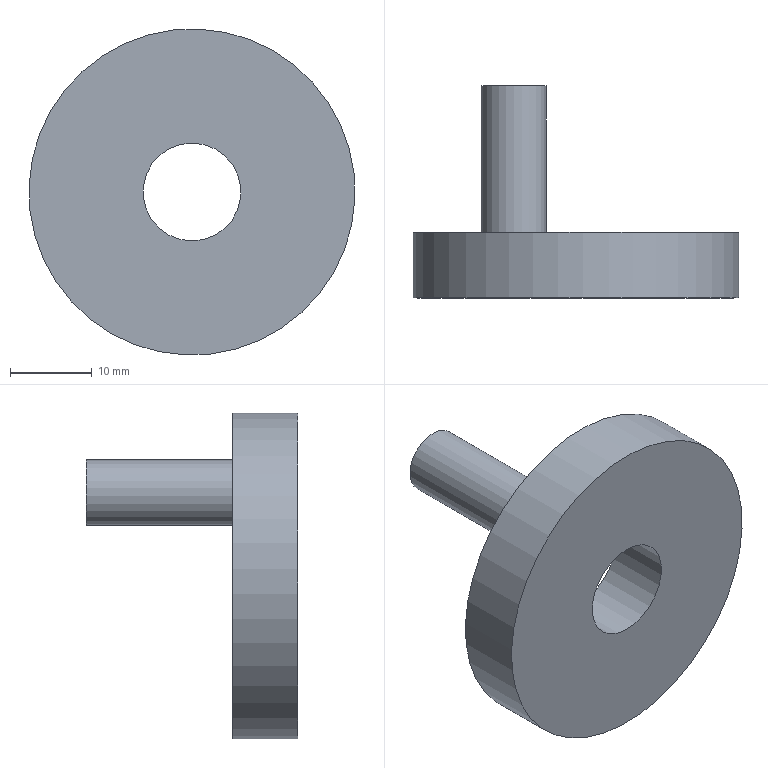Component | NX | CRANK | 1 solid | 6 faces | box 40 x 26 x 40 mm | volume 10053 mm3 | cylinder 3 | plane 3 | commonest cylinder face diameters 40 x1 12 x1 8 x1
STEP:
#1=CARTESIAN_POINT('',(0.,0.,0.));
#2=DIRECTION('',(0.,0.,1.));
#3=DIRECTION('',(1.,0.,0.));
#4=AXIS2_PLACEMENT_3D('',#1,#2,#3);
#5=CARTESIAN_POINT('',(-19.874,30.,-2.24));
#6=VERTEX_POINT('',#5);
#7=CARTESIAN_POINT('',(-0.,30.,0.));
#8=DIRECTION('',(0.,1.,0.));
#9=DIRECTION('',(-0.9937,0.,-0.112));
#10=AXIS2_PLACEMENT_3D('',#7,#8,#9);
#11=CIRCLE('',#10,20.);
#12=CARTESIAN_POINT('',(-0.,30.,0.));
#13=DIRECTION('',(0.,-1.,0.));
#14=DIRECTION('',(0.9937,0.,0.112));
#15=AXIS2_PLACEMENT_3D('',#12,#13,#14);
#16=CYLINDRICAL_SURFACE('',#15,20.);
#17=CARTESIAN_POINT('',(9.425,0.));
#18=DIRECTION('',(-1.,0.));
#19=VECTOR('',#18,1.);
#20=LINE('',#17,#19);
#21=(GEOMETRIC_REPRESENTATION_CONTEXT(2)PARAMETRIC_REPRESENTATION_CONTEXT()REPRESENTATION_CONTEXT('',''));
#22=DEFINITIONAL_REPRESENTATION('',(#20),#21);
#23=PCURVE('',#16,#22);
#24=CARTESIAN_POINT('',(-0.,30.,0.));
#25=DIRECTION('',(0.,1.,0.));
#26=DIRECTION('',(-0.9937,0.,-0.112));
#27=AXIS2_PLACEMENT_3D('',#24,#25,#26);
#28=PLANE('',#27);
#29=CARTESIAN_POINT('',(0.,0.));
#30=DIRECTION('',(1.,0.));
#31=AXIS2_PLACEMENT_2D('',#29,#30);
#32=CIRCLE('',#31,20.);
#33=(GEOMETRIC_REPRESENTATION_CONTEXT(2)PARAMETRIC_REPRESENTATION_CONTEXT()REPRESENTATION_CONTEXT('',''));
#34=DEFINITIONAL_REPRESENTATION('',(#32),#33);
#35=PCURVE('',#28,#34);
#36=SURFACE_CURVE('',#11,(#23,#35),.PCURVE_S1.);
#37=EDGE_CURVE('',#6,#6,#36,.T.);
#38=ORIENTED_EDGE('',*,*,#37,.F.);
#39=CARTESIAN_POINT('',(-19.874,22.,-2.24));
#40=VERTEX_POINT('',#39);
#41=CARTESIAN_POINT('',(-19.874,30.,-2.24));
#42=CARTESIAN_POINT('',(-19.874,22.,-2.24));
#43=B_SPLINE_CURVE_WITH_KNOTS('',1,(#41,#42),.UNSPECIFIED.,.F.,.F.,(2,2),(0.,8.),.PIECEWISE_BEZIER_KNOTS.);
#44=CARTESIAN_POINT('',(9.425,0.));
#45=DIRECTION('',(0.,1.));
#46=VECTOR('',#45,1.);
#47=LINE('',#44,#46);
#48=(GEOMETRIC_REPRESENTATION_CONTEXT(2)PARAMETRIC_REPRESENTATION_CONTEXT()REPRESENTATION_CONTEXT('',''));
#49=DEFINITIONAL_REPRESENTATION('',(#47),#48);
#50=PCURVE('',#16,#49);
#51=CARTESIAN_POINT('',(3.142,0.));
#52=DIRECTION('',(0.,1.));
#53=VECTOR('',#52,1.);
#54=LINE('',#51,#53);
#55=(GEOMETRIC_REPRESENTATION_CONTEXT(2)PARAMETRIC_REPRESENTATION_CONTEXT()REPRESENTATION_CONTEXT('',''));
#56=DEFINITIONAL_REPRESENTATION('',(#54),#55);
#57=PCURVE('',#16,#56);
#58=SEAM_CURVE('',#43,(#50,#57),.PCURVE_S1.);
#59=EDGE_CURVE('',#6,#40,#58,.T.);
#60=ORIENTED_EDGE('',*,*,#59,.T.);
#61=CARTESIAN_POINT('',(-0.,22.,0.));
#62=DIRECTION('',(0.,1.,0.));
#63=DIRECTION('',(-0.9937,0.,-0.112));
#64=AXIS2_PLACEMENT_3D('',#61,#62,#63);
#65=CIRCLE('',#64,20.);
#66=CARTESIAN_POINT('',(9.425,8.));
#67=DIRECTION('',(-1.,0.));
#68=VECTOR('',#67,1.);
#69=LINE('',#66,#68);
#70=(GEOMETRIC_REPRESENTATION_CONTEXT(2)PARAMETRIC_REPRESENTATION_CONTEXT()REPRESENTATION_CONTEXT('',''));
#71=DEFINITIONAL_REPRESENTATION('',(#69),#70);
#72=PCURVE('',#16,#71);
#73=CARTESIAN_POINT('',(-0.,22.,0.));
#74=DIRECTION('',(0.,1.,0.));
#75=DIRECTION('',(-0.9937,0.,-0.112));
#76=AXIS2_PLACEMENT_3D('',#73,#74,#75);
#77=PLANE('',#76);
#78=CARTESIAN_POINT('',(0.,0.));
#79=DIRECTION('',(1.,0.));
#80=AXIS2_PLACEMENT_2D('',#78,#79);
#81=CIRCLE('',#80,20.);
#82=(GEOMETRIC_REPRESENTATION_CONTEXT(2)PARAMETRIC_REPRESENTATION_CONTEXT()REPRESENTATION_CONTEXT('',''));
#83=DEFINITIONAL_REPRESENTATION('',(#81),#82);
#84=PCURVE('',#77,#83);
#85=SURFACE_CURVE('',#65,(#72,#84),.PCURVE_S1.);
#86=EDGE_CURVE('',#40,#40,#85,.T.);
#87=ORIENTED_EDGE('',*,*,#86,.T.);
#88=ORIENTED_EDGE('',*,*,#59,.F.);
#89=EDGE_LOOP('',(#38,#60,#87,#88));
#90=FACE_BOUND('',#89,.T.);
#91=ADVANCED_FACE('',(#90),#16,.T.);
#92=CARTESIAN_POINT('',(-5.962,30.,-0.672));
#93=VERTEX_POINT('',#92);
#94=CARTESIAN_POINT('',(-0.,30.,0.));
#95=DIRECTION('',(0.,1.,0.));
#96=DIRECTION('',(-0.9937,0.,-0.112));
#97=AXIS2_PLACEMENT_3D('',#94,#95,#96);
#98=CIRCLE('',#97,6.);
#99=CARTESIAN_POINT('',(-0.,30.,0.));
#100=DIRECTION('',(0.,-1.,0.));
#101=DIRECTION('',(0.9937,0.,0.112));
#102=AXIS2_PLACEMENT_3D('',#99,#100,#101);
#103=CYLINDRICAL_SURFACE('',#102,6.);
#104=CARTESIAN_POINT('',(9.425,0.));
#105=DIRECTION('',(-1.,0.));
#106=VECTOR('',#105,1.);
#107=LINE('',#104,#106);
#108=(GEOMETRIC_REPRESENTATION_CONTEXT(2)PARAMETRIC_REPRESENTATION_CONTEXT()REPRESENTATION_CONTEXT('',''));
#109=DEFINITIONAL_REPRESENTATION('',(#107),#108);
#110=PCURVE('',#103,#109);
#111=CARTESIAN_POINT('',(0.,0.));
#112=DIRECTION('',(1.,0.));
#113=AXIS2_PLACEMENT_2D('',#111,#112);
#114=CIRCLE('',#113,6.);
#115=(GEOMETRIC_REPRESENTATION_CONTEXT(2)PARAMETRIC_REPRESENTATION_CONTEXT()REPRESENTATION_CONTEXT('',''));
#116=DEFINITIONAL_REPRESENTATION('',(#114),#115);
#117=PCURVE('',#28,#116);
#118=SURFACE_CURVE('',#98,(#110,#117),.PCURVE_S1.);
#119=EDGE_CURVE('',#93,#93,#118,.T.);
#120=ORIENTED_EDGE('',*,*,#119,.F.);
#121=CARTESIAN_POINT('',(-5.962,22.,-0.672));
#122=VERTEX_POINT('',#121);
#123=CARTESIAN_POINT('',(-5.962,30.,-0.672));
#124=CARTESIAN_POINT('',(-5.962,22.,-0.672));
#125=B_SPLINE_CURVE_WITH_KNOTS('',1,(#123,#124),.UNSPECIFIED.,.F.,.F.,(2,2),(0.,8.),.PIECEWISE_BEZIER_KNOTS.);
#126=CARTESIAN_POINT('',(9.425,0.));
#127=DIRECTION('',(0.,1.));
#128=VECTOR('',#127,1.);
#129=LINE('',#126,#128);
#130=(GEOMETRIC_REPRESENTATION_CONTEXT(2)PARAMETRIC_REPRESENTATION_CONTEXT()REPRESENTATION_CONTEXT('',''));
#131=DEFINITIONAL_REPRESENTATION('',(#129),#130);
#132=PCURVE('',#103,#131);
#133=CARTESIAN_POINT('',(3.142,0.));
#134=DIRECTION('',(0.,1.));
#135=VECTOR('',#134,1.);
#136=LINE('',#133,#135);
#137=(GEOMETRIC_REPRESENTATION_CONTEXT(2)PARAMETRIC_REPRESENTATION_CONTEXT()REPRESENTATION_CONTEXT('',''));
#138=DEFINITIONAL_REPRESENTATION('',(#136),#137);
#139=PCURVE('',#103,#138);
#140=SEAM_CURVE('',#125,(#132,#139),.PCURVE_S1.);
#141=EDGE_CURVE('',#93,#122,#140,.T.);
#142=ORIENTED_EDGE('',*,*,#141,.T.);
#143=CARTESIAN_POINT('',(-0.,22.,0.));
#144=DIRECTION('',(0.,1.,0.));
#145=DIRECTION('',(-0.9937,0.,-0.112));
#146=AXIS2_PLACEMENT_3D('',#143,#144,#145);
#147=CIRCLE('',#146,6.);
#148=CARTESIAN_POINT('',(9.425,8.));
#149=DIRECTION('',(-1.,0.));
#150=VECTOR('',#149,1.);
#151=LINE('',#148,#150);
#152=(GEOMETRIC_REPRESENTATION_CONTEXT(2)PARAMETRIC_REPRESENTATION_CONTEXT()REPRESENTATION_CONTEXT('',''));
#153=DEFINITIONAL_REPRESENTATION('',(#151),#152);
#154=PCURVE('',#103,#153);
#155=CARTESIAN_POINT('',(0.,0.));
#156=DIRECTION('',(1.,0.));
#157=AXIS2_PLACEMENT_2D('',#155,#156);
#158=CIRCLE('',#157,6.);
#159=(GEOMETRIC_REPRESENTATION_CONTEXT(2)PARAMETRIC_REPRESENTATION_CONTEXT()REPRESENTATION_CONTEXT('',''));
#160=DEFINITIONAL_REPRESENTATION('',(#158),#159);
#161=PCURVE('',#77,#160);
#162=SURFACE_CURVE('',#147,(#154,#161),.PCURVE_S1.);
#163=EDGE_CURVE('',#122,#122,#162,.T.);
#164=ORIENTED_EDGE('',*,*,#163,.T.);
#165=ORIENTED_EDGE('',*,*,#141,.F.);
#166=EDGE_LOOP('',(#120,#142,#164,#165));
#167=FACE_BOUND('',#166,.F.);
#168=ADVANCED_FACE('',(#167),#103,.F.);
#169=CARTESIAN_POINT('',(-11.615,30.,9.787));
#170=VERTEX_POINT('',#169);
#171=CARTESIAN_POINT('',(-7.64,30.,10.235));
#172=DIRECTION('',(0.,1.,0.));
#173=DIRECTION('',(-0.9937,0.,-0.112));
#174=AXIS2_PLACEMENT_3D('',#171,#172,#173);
#175=CIRCLE('',#174,4.);
#176=CARTESIAN_POINT('',(6.446,11.027));
#177=DIRECTION('',(1.,0.));
#178=AXIS2_PLACEMENT_2D('',#176,#177);
#179=CIRCLE('',#178,4.);
#180=(GEOMETRIC_REPRESENTATION_CONTEXT(2)PARAMETRIC_REPRESENTATION_CONTEXT()REPRESENTATION_CONTEXT('',''));
#181=DEFINITIONAL_REPRESENTATION('',(#179),#180);
#182=PCURVE('',#28,#181);
#183=CARTESIAN_POINT('',(-7.64,48.,10.235));
#184=DIRECTION('',(0.,-1.,0.));
#185=DIRECTION('',(0.9937,0.,0.112));
#186=AXIS2_PLACEMENT_3D('',#183,#184,#185);
#187=CYLINDRICAL_SURFACE('',#186,4.);
#188=CARTESIAN_POINT('',(9.425,18.));
#189=DIRECTION('',(-1.,0.));
#190=VECTOR('',#189,1.);
#191=LINE('',#188,#190);
#192=(GEOMETRIC_REPRESENTATION_CONTEXT(2)PARAMETRIC_REPRESENTATION_CONTEXT()REPRESENTATION_CONTEXT('',''));
#193=DEFINITIONAL_REPRESENTATION('',(#191),#192);
#194=PCURVE('',#187,#193);
#195=SURFACE_CURVE('',#175,(#182,#194),.PCURVE_S1.);
#196=EDGE_CURVE('',#170,#170,#195,.T.);
#197=ORIENTED_EDGE('',*,*,#196,.F.);
#198=EDGE_LOOP('',(#197));
#199=FACE_BOUND('',#198,.T.);
#200=ORIENTED_EDGE('',*,*,#37,.T.);
#201=EDGE_LOOP('',(#200));
#202=FACE_BOUND('',#201,.T.);
#203=ORIENTED_EDGE('',*,*,#119,.F.);
#204=EDGE_LOOP('',(#203));
#205=FACE_BOUND('',#204,.T.);
#206=ADVANCED_FACE('',(#199,#202,#205),#28,.T.);
#207=ORIENTED_EDGE('',*,*,#86,.F.);
#208=EDGE_LOOP('',(#207));
#209=FACE_BOUND('',#208,.T.);
#210=ORIENTED_EDGE('',*,*,#163,.T.);
#211=EDGE_LOOP('',(#210));
#212=FACE_BOUND('',#211,.T.);
#213=ADVANCED_FACE('',(#209,#212),#77,.F.);
#214=CARTESIAN_POINT('',(-11.615,48.,9.787));
#215=VERTEX_POINT('',#214);
#216=CARTESIAN_POINT('',(-7.64,48.,10.235));
#217=DIRECTION('',(0.,1.,0.));
#218=DIRECTION('',(-0.9937,0.,-0.112));
#219=AXIS2_PLACEMENT_3D('',#216,#217,#218);
#220=CIRCLE('',#219,4.);
#221=CARTESIAN_POINT('',(9.425,0.));
#222=DIRECTION('',(-1.,0.));
#223=VECTOR('',#222,1.);
#224=LINE('',#221,#223);
#225=(GEOMETRIC_REPRESENTATION_CONTEXT(2)PARAMETRIC_REPRESENTATION_CONTEXT()REPRESENTATION_CONTEXT('',''));
#226=DEFINITIONAL_REPRESENTATION('',(#224),#225);
#227=PCURVE('',#187,#226);
#228=CARTESIAN_POINT('',(-7.64,48.,10.235));
#229=DIRECTION('',(0.,1.,0.));
#230=DIRECTION('',(-0.9937,0.,-0.112));
#231=AXIS2_PLACEMENT_3D('',#228,#229,#230);
#232=PLANE('',#231);
#233=CARTESIAN_POINT('',(0.,0.));
#234=DIRECTION('',(1.,0.));
#235=AXIS2_PLACEMENT_2D('',#233,#234);
#236=CIRCLE('',#235,4.);
#237=(GEOMETRIC_REPRESENTATION_CONTEXT(2)PARAMETRIC_REPRESENTATION_CONTEXT()REPRESENTATION_CONTEXT('',''));
#238=DEFINITIONAL_REPRESENTATION('',(#236),#237);
#239=PCURVE('',#232,#238);
#240=SURFACE_CURVE('',#220,(#227,#239),.PCURVE_S1.);
#241=EDGE_CURVE('',#215,#215,#240,.T.);
#242=ORIENTED_EDGE('',*,*,#241,.F.);
#243=CARTESIAN_POINT('',(-11.615,48.,9.787));
#244=CARTESIAN_POINT('',(-11.615,30.,9.787));
#245=B_SPLINE_CURVE_WITH_KNOTS('',1,(#243,#244),.UNSPECIFIED.,.F.,.F.,(2,2),(0.,18.),.PIECEWISE_BEZIER_KNOTS.);
#246=CARTESIAN_POINT('',(9.425,0.));
#247=DIRECTION('',(0.,1.));
#248=VECTOR('',#247,1.);
#249=LINE('',#246,#248);
#250=(GEOMETRIC_REPRESENTATION_CONTEXT(2)PARAMETRIC_REPRESENTATION_CONTEXT()REPRESENTATION_CONTEXT('',''));
#251=DEFINITIONAL_REPRESENTATION('',(#249),#250);
#252=PCURVE('',#187,#251);
#253=CARTESIAN_POINT('',(3.142,0.));
#254=DIRECTION('',(0.,1.));
#255=VECTOR('',#254,1.);
#256=LINE('',#253,#255);
#257=(GEOMETRIC_REPRESENTATION_CONTEXT(2)PARAMETRIC_REPRESENTATION_CONTEXT()REPRESENTATION_CONTEXT('',''));
#258=DEFINITIONAL_REPRESENTATION('',(#256),#257);
#259=PCURVE('',#187,#258);
#260=SEAM_CURVE('',#245,(#252,#259),.PCURVE_S1.);
#261=EDGE_CURVE('',#215,#170,#260,.T.);
#262=ORIENTED_EDGE('',*,*,#261,.T.);
#263=ORIENTED_EDGE('',*,*,#196,.T.);
#264=ORIENTED_EDGE('',*,*,#261,.F.);
#265=EDGE_LOOP('',(#242,#262,#263,#264));
#266=FACE_BOUND('',#265,.T.);
#267=ADVANCED_FACE('',(#266),#187,.T.);
#268=ORIENTED_EDGE('',*,*,#241,.T.);
#269=EDGE_LOOP('',(#268));
#270=FACE_BOUND('',#269,.T.);
#271=ADVANCED_FACE('',(#270),#232,.T.);
#272=CLOSED_SHELL('',(#91,#168,#206,#213,#267,#271));
#273=MANIFOLD_SOLID_BREP('',#272);
#274=(LENGTH_UNIT()NAMED_UNIT(*)SI_UNIT(.MILLI.,.METRE.));
#275=UNCERTAINTY_MEASURE_WITH_UNIT(LENGTH_MEASURE(0.00001),#274,'','');
#276=(NAMED_UNIT(*)PLANE_ANGLE_UNIT()SI_UNIT($,.RADIAN.));
#277=(NAMED_UNIT(*)SI_UNIT($,.STERADIAN.)SOLID_ANGLE_UNIT());
#278=(GEOMETRIC_REPRESENTATION_CONTEXT(3)GLOBAL_UNCERTAINTY_ASSIGNED_CONTEXT((#275))GLOBAL_UNIT_ASSIGNED_CONTEXT((#274,#276,#277))REPRESENTATION_CONTEXT('',''));
#279=ADVANCED_BREP_SHAPE_REPRESENTATION('',(#4,#273),#278);